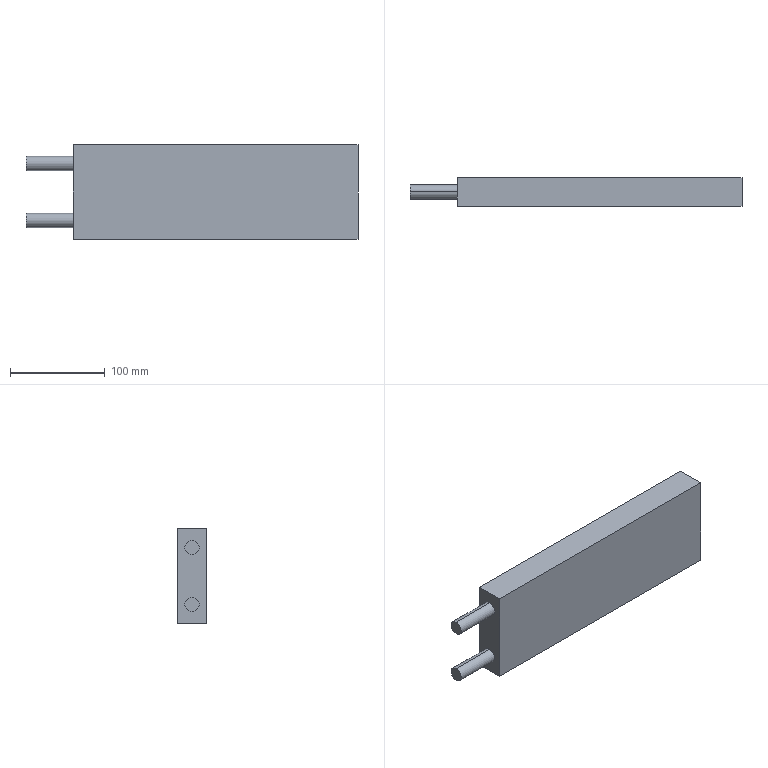Component | SolidWorks | HeatingBlock.1-1 | 1 solid | 12 faces | box 350 x 30 x 100 mm | volume 917671 mm3 | plane 8 | cylinder 4 | commonest cylinder face diameters 15 x4
build123d program:
from build123d import *

# Parameters (mm, degrees)
SKETCH1_W           = 100
SKETCH1_H           = 30
BOSS_EXTRUDE1_DEPTH = 150
SKETCH2_R           = 7.5
BOSS_EXTRUDE2_DEPTH = 50


with BuildPart() as part:
    # Sketch1 → Boss-Extrude1 (new, symmetric)
    with BuildSketch(Plane.XY):
        Rectangle(SKETCH1_W, SKETCH1_H)
    extrude(amount=BOSS_EXTRUDE1_DEPTH, both=True)

    # Sketch2 → Boss-Extrude2 (add)
    with BuildSketch(Plane.XY.offset(150)):
        with Locations((-30, 0)):
            Circle(SKETCH2_R)
        with Locations((30, 0)):
            Circle(SKETCH2_R)
    extrude(amount=BOSS_EXTRUDE2_DEPTH)


solid = part.part

# Placed as in the assembly
solid = solid.moved(Location((512, 118.5, 0), (0, -90, 0)))
STEP:
#1=CARTESIAN_POINT('',(12.283,4.665,1.476));
#2=VERTEX_POINT('',#1);
#3=CARTESIAN_POINT('',(12.283,4.665,0.8858));
#4=VERTEX_POINT('',#3);
#5=CARTESIAN_POINT('',(12.283,4.665,1.181));
#6=DIRECTION('',(-1.,0.,-0.));
#7=DIRECTION('',(0.,0.,1.));
#8=AXIS2_PLACEMENT_3D('',#5,#6,#7);
#9=CIRCLE('',#8,0.2953);
#10=EDGE_CURVE('',#2,#4,#9,.T.);
#11=ORIENTED_EDGE('',*,*,#10,.F.);
#12=CARTESIAN_POINT('',(14.252,4.665,1.476));
#13=VERTEX_POINT('',#12);
#14=CARTESIAN_POINT('',(12.283,4.665,1.476));
#15=DIRECTION('',(1.,-0.,0.));
#16=VECTOR('',#15,39.37);
#17=LINE('',#14,#16);
#18=EDGE_CURVE('',#2,#13,#17,.T.);
#19=ORIENTED_EDGE('',*,*,#18,.T.);
#20=CARTESIAN_POINT('',(14.252,4.665,0.8858));
#21=VERTEX_POINT('',#20);
#22=CARTESIAN_POINT('',(14.252,4.665,1.181));
#23=DIRECTION('',(-1.,0.,-0.));
#24=DIRECTION('',(0.,0.,1.));
#25=AXIS2_PLACEMENT_3D('',#22,#23,#24);
#26=CIRCLE('',#25,0.2953);
#27=EDGE_CURVE('',#13,#21,#26,.T.);
#28=ORIENTED_EDGE('',*,*,#27,.T.);
#29=CARTESIAN_POINT('',(12.283,4.665,0.8858));
#30=DIRECTION('',(1.,-0.,0.));
#31=VECTOR('',#30,39.37);
#32=LINE('',#29,#31);
#33=EDGE_CURVE('',#4,#21,#32,.T.);
#34=ORIENTED_EDGE('',*,*,#33,.F.);
#35=EDGE_LOOP('',(#11,#19,#28,#34));
#36=FACE_OUTER_BOUND('',#35,.T.);
#37=CARTESIAN_POINT('',(12.283,4.665,1.181));
#38=DIRECTION('',(1.,-0.,0.));
#39=DIRECTION('',(0.,0.,-1.));
#40=AXIS2_PLACEMENT_3D('',#37,#38,#39);
#41=CYLINDRICAL_SURFACE('',#40,0.2953);
#42=ADVANCED_FACE('',(#36),#41,.T.);
#43=CARTESIAN_POINT('',(12.283,4.665,-0.8858));
#44=VERTEX_POINT('',#43);
#45=CARTESIAN_POINT('',(12.283,4.665,-1.476));
#46=VERTEX_POINT('',#45);
#47=CARTESIAN_POINT('',(12.283,4.665,-1.181));
#48=DIRECTION('',(-1.,0.,-0.));
#49=DIRECTION('',(0.,0.,1.));
#50=AXIS2_PLACEMENT_3D('',#47,#48,#49);
#51=CIRCLE('',#50,0.2953);
#52=EDGE_CURVE('',#44,#46,#51,.T.);
#53=ORIENTED_EDGE('',*,*,#52,.F.);
#54=CARTESIAN_POINT('',(14.252,4.665,-0.8858));
#55=VERTEX_POINT('',#54);
#56=CARTESIAN_POINT('',(12.283,4.665,-0.8858));
#57=DIRECTION('',(1.,-0.,0.));
#58=VECTOR('',#57,39.37);
#59=LINE('',#56,#58);
#60=EDGE_CURVE('',#44,#55,#59,.T.);
#61=ORIENTED_EDGE('',*,*,#60,.T.);
#62=CARTESIAN_POINT('',(14.252,4.665,-1.476));
#63=VERTEX_POINT('',#62);
#64=CARTESIAN_POINT('',(14.252,4.665,-1.181));
#65=DIRECTION('',(-1.,0.,-0.));
#66=DIRECTION('',(0.,0.,1.));
#67=AXIS2_PLACEMENT_3D('',#64,#65,#66);
#68=CIRCLE('',#67,0.2953);
#69=EDGE_CURVE('',#55,#63,#68,.T.);
#70=ORIENTED_EDGE('',*,*,#69,.T.);
#71=CARTESIAN_POINT('',(12.283,4.665,-1.476));
#72=DIRECTION('',(1.,-0.,0.));
#73=VECTOR('',#72,39.37);
#74=LINE('',#71,#73);
#75=EDGE_CURVE('',#46,#63,#74,.T.);
#76=ORIENTED_EDGE('',*,*,#75,.F.);
#77=EDGE_LOOP('',(#53,#61,#70,#76));
#78=FACE_OUTER_BOUND('',#77,.T.);
#79=CARTESIAN_POINT('',(12.283,4.665,-1.181));
#80=DIRECTION('',(1.,-0.,0.));
#81=DIRECTION('',(0.,0.,-1.));
#82=AXIS2_PLACEMENT_3D('',#79,#80,#81);
#83=CYLINDRICAL_SURFACE('',#82,0.2953);
#84=ADVANCED_FACE('',(#78),#83,.T.);
#85=CARTESIAN_POINT('',(14.252,4.665,-1.181));
#86=DIRECTION('',(-1.,0.,-0.));
#87=DIRECTION('',(0.,0.,1.));
#88=AXIS2_PLACEMENT_3D('',#85,#86,#87);
#89=CIRCLE('',#88,0.2953);
#90=EDGE_CURVE('',#63,#55,#89,.T.);
#91=ORIENTED_EDGE('',*,*,#90,.F.);
#92=ORIENTED_EDGE('',*,*,#69,.F.);
#93=EDGE_LOOP('',(#91,#92));
#94=FACE_BOUND('',#93,.T.);
#95=CARTESIAN_POINT('',(14.252,4.075,1.969));
#96=VERTEX_POINT('',#95);
#97=CARTESIAN_POINT('',(14.252,5.256,1.969));
#98=VERTEX_POINT('',#97);
#99=CARTESIAN_POINT('',(14.252,5.256,1.969));
#100=DIRECTION('',(0.,1.,-0.));
#101=VECTOR('',#100,39.37);
#102=LINE('',#99,#101);
#103=EDGE_CURVE('',#96,#98,#102,.T.);
#104=ORIENTED_EDGE('',*,*,#103,.T.);
#105=CARTESIAN_POINT('',(14.252,5.256,-1.969));
#106=VERTEX_POINT('',#105);
#107=CARTESIAN_POINT('',(14.252,5.256,-1.969));
#108=DIRECTION('',(0.,-0.,-1.));
#109=VECTOR('',#108,39.37);
#110=LINE('',#107,#109);
#111=EDGE_CURVE('',#98,#106,#110,.T.);
#112=ORIENTED_EDGE('',*,*,#111,.T.);
#113=CARTESIAN_POINT('',(14.252,4.075,-1.969));
#114=VERTEX_POINT('',#113);
#115=CARTESIAN_POINT('',(14.252,5.256,-1.969));
#116=DIRECTION('',(-0.,-1.,0.));
#117=VECTOR('',#116,39.37);
#118=LINE('',#115,#117);
#119=EDGE_CURVE('',#106,#114,#118,.T.);
#120=ORIENTED_EDGE('',*,*,#119,.T.);
#121=CARTESIAN_POINT('',(14.252,4.075,-1.969));
#122=DIRECTION('',(-0.,0.,1.));
#123=VECTOR('',#122,39.37);
#124=LINE('',#121,#123);
#125=EDGE_CURVE('',#114,#96,#124,.T.);
#126=ORIENTED_EDGE('',*,*,#125,.T.);
#127=EDGE_LOOP('',(#104,#112,#120,#126));
#128=FACE_OUTER_BOUND('',#127,.T.);
#129=CARTESIAN_POINT('',(14.252,4.665,1.181));
#130=DIRECTION('',(-1.,0.,-0.));
#131=DIRECTION('',(0.,0.,1.));
#132=AXIS2_PLACEMENT_3D('',#129,#130,#131);
#133=CIRCLE('',#132,0.2953);
#134=EDGE_CURVE('',#21,#13,#133,.T.);
#135=ORIENTED_EDGE('',*,*,#134,.F.);
#136=ORIENTED_EDGE('',*,*,#27,.F.);
#137=EDGE_LOOP('',(#135,#136));
#138=FACE_BOUND('',#137,.T.);
#139=CARTESIAN_POINT('',(14.252,4.075,1.969));
#140=DIRECTION('',(-1.,0.,-0.));
#141=DIRECTION('',(-0.,0.,1.));
#142=AXIS2_PLACEMENT_3D('',#139,#140,#141);
#143=PLANE('',#142);
#144=ADVANCED_FACE('',(#94,#128,#138),#143,.T.);
#145=CARTESIAN_POINT('',(26.063,4.075,1.969));
#146=VERTEX_POINT('',#145);
#147=CARTESIAN_POINT('',(26.063,5.256,1.969));
#148=VERTEX_POINT('',#147);
#149=CARTESIAN_POINT('',(26.063,5.256,1.969));
#150=DIRECTION('',(0.,1.,-0.));
#151=VECTOR('',#150,39.37);
#152=LINE('',#149,#151);
#153=EDGE_CURVE('',#146,#148,#152,.T.);
#154=ORIENTED_EDGE('',*,*,#153,.T.);
#155=CARTESIAN_POINT('',(14.252,5.256,1.969));
#156=DIRECTION('',(1.,-0.,0.));
#157=VECTOR('',#156,39.37);
#158=LINE('',#155,#157);
#159=EDGE_CURVE('',#98,#148,#158,.T.);
#160=ORIENTED_EDGE('',*,*,#159,.F.);
#161=ORIENTED_EDGE('',*,*,#103,.F.);
#162=CARTESIAN_POINT('',(14.252,4.075,1.969));
#163=DIRECTION('',(1.,-0.,0.));
#164=VECTOR('',#163,39.37);
#165=LINE('',#162,#164);
#166=EDGE_CURVE('',#96,#146,#165,.T.);
#167=ORIENTED_EDGE('',*,*,#166,.T.);
#168=EDGE_LOOP('',(#154,#160,#161,#167));
#169=FACE_OUTER_BOUND('',#168,.T.);
#170=CARTESIAN_POINT('',(14.252,5.256,1.969));
#171=DIRECTION('',(0.,-0.,-1.));
#172=DIRECTION('',(-1.,0.,-0.));
#173=AXIS2_PLACEMENT_3D('',#170,#171,#172);
#174=PLANE('',#173);
#175=ADVANCED_FACE('',(#169),#174,.F.);
#176=CARTESIAN_POINT('',(26.063,5.256,-1.969));
#177=VERTEX_POINT('',#176);
#178=CARTESIAN_POINT('',(26.063,5.256,-1.969));
#179=DIRECTION('',(0.,-0.,-1.));
#180=VECTOR('',#179,39.37);
#181=LINE('',#178,#180);
#182=EDGE_CURVE('',#148,#177,#181,.T.);
#183=ORIENTED_EDGE('',*,*,#182,.T.);
#184=CARTESIAN_POINT('',(14.252,5.256,-1.969));
#185=DIRECTION('',(1.,-0.,0.));
#186=VECTOR('',#185,39.37);
#187=LINE('',#184,#186);
#188=EDGE_CURVE('',#106,#177,#187,.T.);
#189=ORIENTED_EDGE('',*,*,#188,.F.);
#190=ORIENTED_EDGE('',*,*,#111,.F.);
#191=ORIENTED_EDGE('',*,*,#159,.T.);
#192=EDGE_LOOP('',(#183,#189,#190,#191));
#193=FACE_OUTER_BOUND('',#192,.T.);
#194=CARTESIAN_POINT('',(14.252,5.256,-1.969));
#195=DIRECTION('',(-0.,-1.,0.));
#196=DIRECTION('',(1.,-0.,0.));
#197=AXIS2_PLACEMENT_3D('',#194,#195,#196);
#198=PLANE('',#197);
#199=ADVANCED_FACE('',(#193),#198,.F.);
#200=CARTESIAN_POINT('',(26.063,4.075,-1.969));
#201=VERTEX_POINT('',#200);
#202=CARTESIAN_POINT('',(26.063,5.256,-1.969));
#203=DIRECTION('',(-0.,-1.,0.));
#204=VECTOR('',#203,39.37);
#205=LINE('',#202,#204);
#206=EDGE_CURVE('',#177,#201,#205,.T.);
#207=ORIENTED_EDGE('',*,*,#206,.T.);
#208=CARTESIAN_POINT('',(14.252,4.075,-1.969));
#209=DIRECTION('',(1.,-0.,0.));
#210=VECTOR('',#209,39.37);
#211=LINE('',#208,#210);
#212=EDGE_CURVE('',#114,#201,#211,.T.);
#213=ORIENTED_EDGE('',*,*,#212,.F.);
#214=ORIENTED_EDGE('',*,*,#119,.F.);
#215=ORIENTED_EDGE('',*,*,#188,.T.);
#216=EDGE_LOOP('',(#207,#213,#214,#215));
#217=FACE_OUTER_BOUND('',#216,.T.);
#218=CARTESIAN_POINT('',(14.252,5.256,-1.969));
#219=DIRECTION('',(-0.,0.,1.));
#220=DIRECTION('',(1.,-0.,0.));
#221=AXIS2_PLACEMENT_3D('',#218,#219,#220);
#222=PLANE('',#221);
#223=ADVANCED_FACE('',(#217),#222,.F.);
#224=CARTESIAN_POINT('',(26.063,4.075,-1.969));
#225=DIRECTION('',(-0.,0.,1.));
#226=VECTOR('',#225,39.37);
#227=LINE('',#224,#226);
#228=EDGE_CURVE('',#201,#146,#227,.T.);
#229=ORIENTED_EDGE('',*,*,#228,.T.);
#230=ORIENTED_EDGE('',*,*,#166,.F.);
#231=ORIENTED_EDGE('',*,*,#125,.F.);
#232=ORIENTED_EDGE('',*,*,#212,.T.);
#233=EDGE_LOOP('',(#229,#230,#231,#232));
#234=FACE_OUTER_BOUND('',#233,.T.);
#235=CARTESIAN_POINT('',(14.252,4.075,-1.969));
#236=DIRECTION('',(0.,1.,-0.));
#237=DIRECTION('',(-1.,0.,-0.));
#238=AXIS2_PLACEMENT_3D('',#235,#236,#237);
#239=PLANE('',#238);
#240=ADVANCED_FACE('',(#234),#239,.F.);
#241=ORIENTED_EDGE('',*,*,#153,.F.);
#242=ORIENTED_EDGE('',*,*,#228,.F.);
#243=ORIENTED_EDGE('',*,*,#206,.F.);
#244=ORIENTED_EDGE('',*,*,#182,.F.);
#245=EDGE_LOOP('',(#241,#242,#243,#244));
#246=FACE_OUTER_BOUND('',#245,.T.);
#247=CARTESIAN_POINT('',(26.063,4.075,1.969));
#248=DIRECTION('',(-1.,0.,-0.));
#249=DIRECTION('',(-0.,0.,1.));
#250=AXIS2_PLACEMENT_3D('',#247,#248,#249);
#251=PLANE('',#250);
#252=ADVANCED_FACE('',(#246),#251,.F.);
#253=ORIENTED_EDGE('',*,*,#60,.F.);
#254=CARTESIAN_POINT('',(12.283,4.665,-1.181));
#255=DIRECTION('',(-1.,0.,-0.));
#256=DIRECTION('',(0.,0.,1.));
#257=AXIS2_PLACEMENT_3D('',#254,#255,#256);
#258=CIRCLE('',#257,0.2953);
#259=EDGE_CURVE('',#46,#44,#258,.T.);
#260=ORIENTED_EDGE('',*,*,#259,.F.);
#261=ORIENTED_EDGE('',*,*,#75,.T.);
#262=ORIENTED_EDGE('',*,*,#90,.T.);
#263=EDGE_LOOP('',(#253,#260,#261,#262));
#264=FACE_OUTER_BOUND('',#263,.T.);
#265=CARTESIAN_POINT('',(12.283,4.665,-1.181));
#266=DIRECTION('',(1.,-0.,0.));
#267=DIRECTION('',(0.,0.,-1.));
#268=AXIS2_PLACEMENT_3D('',#265,#266,#267);
#269=CYLINDRICAL_SURFACE('',#268,0.2953);
#270=ADVANCED_FACE('',(#264),#269,.T.);
#271=ORIENTED_EDGE('',*,*,#259,.T.);
#272=ORIENTED_EDGE('',*,*,#52,.T.);
#273=EDGE_LOOP('',(#271,#272));
#274=FACE_OUTER_BOUND('',#273,.T.);
#275=CARTESIAN_POINT('',(12.283,4.665,-1.181));
#276=DIRECTION('',(-1.,0.,-0.));
#277=DIRECTION('',(-0.,0.,1.));
#278=AXIS2_PLACEMENT_3D('',#275,#276,#277);
#279=PLANE('',#278);
#280=ADVANCED_FACE('',(#274),#279,.T.);
#281=ORIENTED_EDGE('',*,*,#18,.F.);
#282=CARTESIAN_POINT('',(12.283,4.665,1.181));
#283=DIRECTION('',(-1.,0.,-0.));
#284=DIRECTION('',(0.,0.,1.));
#285=AXIS2_PLACEMENT_3D('',#282,#283,#284);
#286=CIRCLE('',#285,0.2953);
#287=EDGE_CURVE('',#4,#2,#286,.T.);
#288=ORIENTED_EDGE('',*,*,#287,.F.);
#289=ORIENTED_EDGE('',*,*,#33,.T.);
#290=ORIENTED_EDGE('',*,*,#134,.T.);
#291=EDGE_LOOP('',(#281,#288,#289,#290));
#292=FACE_OUTER_BOUND('',#291,.T.);
#293=CARTESIAN_POINT('',(12.283,4.665,1.181));
#294=DIRECTION('',(1.,-0.,0.));
#295=DIRECTION('',(0.,0.,-1.));
#296=AXIS2_PLACEMENT_3D('',#293,#294,#295);
#297=CYLINDRICAL_SURFACE('',#296,0.2953);
#298=ADVANCED_FACE('',(#292),#297,.T.);
#299=ORIENTED_EDGE('',*,*,#287,.T.);
#300=ORIENTED_EDGE('',*,*,#10,.T.);
#301=EDGE_LOOP('',(#299,#300));
#302=FACE_OUTER_BOUND('',#301,.T.);
#303=CARTESIAN_POINT('',(12.283,4.665,1.181));
#304=DIRECTION('',(-1.,0.,-0.));
#305=DIRECTION('',(-0.,0.,1.));
#306=AXIS2_PLACEMENT_3D('',#303,#304,#305);
#307=PLANE('',#306);
#308=ADVANCED_FACE('',(#302),#307,.T.);
#309=CLOSED_SHELL('',(#42,#84,#144,#175,#199,#223,#240,#252,#270,#280,#298,#308));
#310=MANIFOLD_SOLID_BREP('',#309);
#311=CARTESIAN_POINT('',(0.,0.,0.));
#312=DIRECTION('',(0.,0.,1.));
#313=DIRECTION('',(1.,0.,0.));
#314=AXIS2_PLACEMENT_3D('',#311,#312,#313);
#315=(LENGTH_UNIT()NAMED_UNIT(*)SI_UNIT($,.METRE.));
#316=LENGTH_MEASURE_WITH_UNIT(LENGTH_MEASURE(0.0254),#315);
#317=DIMENSIONAL_EXPONENTS(1.,0.,0.,0.,0.,0.,0.);
#318=(CONVERSION_BASED_UNIT('',#316)LENGTH_UNIT()NAMED_UNIT(#317));
#319=UNCERTAINTY_MEASURE_WITH_UNIT(LENGTH_MEASURE(0.00001),#318,'','');
#320=(NAMED_UNIT(*)PLANE_ANGLE_UNIT()SI_UNIT($,.RADIAN.));
#321=(NAMED_UNIT(*)SI_UNIT($,.STERADIAN.)SOLID_ANGLE_UNIT());
#322=(GEOMETRIC_REPRESENTATION_CONTEXT(3)GLOBAL_UNCERTAINTY_ASSIGNED_CONTEXT((#319))GLOBAL_UNIT_ASSIGNED_CONTEXT((#318,#320,#321))REPRESENTATION_CONTEXT('',''));
#323=ADVANCED_BREP_SHAPE_REPRESENTATION('',(#310,#314),#322);
#324=COLOUR_RGB('',0.7922,0.8196,0.9333);
#325=FILL_AREA_STYLE_COLOUR('',#324);
#326=FILL_AREA_STYLE('',(#325));
#327=SURFACE_STYLE_FILL_AREA(#326);
#328=SURFACE_SIDE_STYLE('',(#327));
#329=SURFACE_STYLE_USAGE(.BOTH.,#328);
#330=PRESENTATION_STYLE_ASSIGNMENT((#329));
#331=STYLED_ITEM('',(#330),#310);
#332=PRESENTATION_LAYER_ASSIGNMENT('','',(#331));
#333=(LENGTH_UNIT()NAMED_UNIT(*)SI_UNIT($,.METRE.));
#334=LENGTH_MEASURE_WITH_UNIT(LENGTH_MEASURE(0.0254),#333);
#335=DIMENSIONAL_EXPONENTS(1.,0.,0.,0.,0.,0.,0.);
#336=(CONVERSION_BASED_UNIT('',#334)LENGTH_UNIT()NAMED_UNIT(#335));
#337=UNCERTAINTY_MEASURE_WITH_UNIT(LENGTH_MEASURE(0.00001),#336,'','');
#338=(NAMED_UNIT(*)PLANE_ANGLE_UNIT()SI_UNIT($,.RADIAN.));
#339=(NAMED_UNIT(*)SI_UNIT($,.STERADIAN.)SOLID_ANGLE_UNIT());
#340=(GEOMETRIC_REPRESENTATION_CONTEXT(3)GLOBAL_UNCERTAINTY_ASSIGNED_CONTEXT((#337))GLOBAL_UNIT_ASSIGNED_CONTEXT((#336,#338,#339))REPRESENTATION_CONTEXT('',''));
#341=MECHANICAL_DESIGN_GEOMETRIC_PRESENTATION_REPRESENTATION('',(#331),#340);